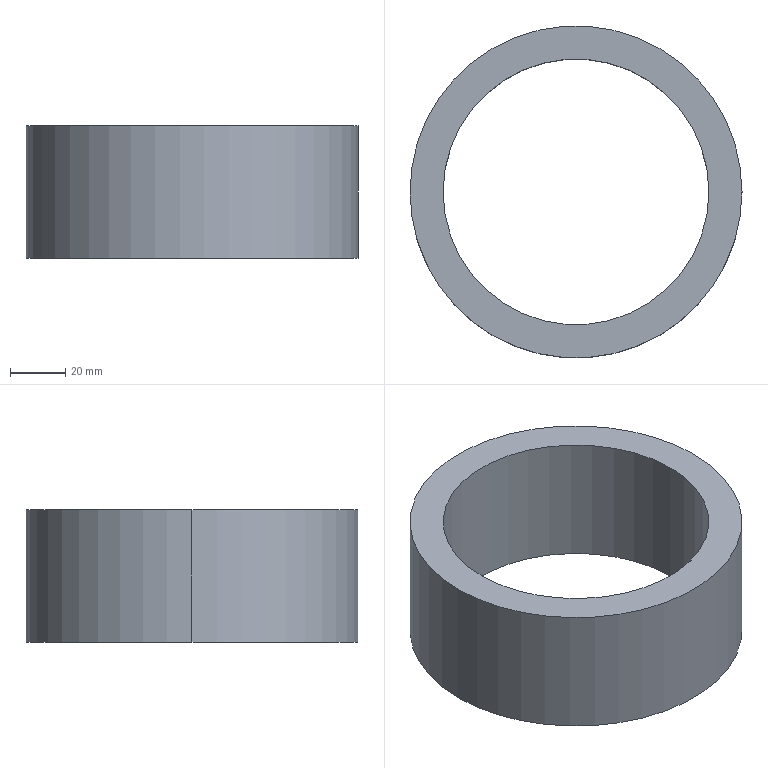Component | SolidWorks | 5-1 | 1 solid | 6 faces | box 120 x 120 x 48 mm | volume 194998 mm3 | cylinder 4 | plane 2 | commonest cylinder face diameters 96.06 x2 120 x2
STEP:
#1=CARTESIAN_POINT('',(1.891,0.,-1.89));
#2=VERTEX_POINT('',#1);
#3=CARTESIAN_POINT('',(1.891,0.,-3.78));
#4=VERTEX_POINT('',#3);
#5=CARTESIAN_POINT('',(1.891,0.,-1.89));
#6=DIRECTION('',(0.,0.,-1.));
#7=VECTOR('',#6,39.37);
#8=LINE('',#5,#7);
#9=EDGE_CURVE('',#2,#4,#8,.T.);
#10=ORIENTED_EDGE('',*,*,#9,.F.);
#11=CARTESIAN_POINT('',(-1.891,0.,-1.89));
#12=VERTEX_POINT('',#11);
#13=CARTESIAN_POINT('',(0.,0.,-1.89));
#14=DIRECTION('',(0.,0.,1.));
#15=DIRECTION('',(1.,0.,0.));
#16=AXIS2_PLACEMENT_3D('',#13,#14,#15);
#17=CIRCLE('',#16,1.891);
#18=EDGE_CURVE('',#2,#12,#17,.T.);
#19=ORIENTED_EDGE('',*,*,#18,.T.);
#20=CARTESIAN_POINT('',(-1.891,0.,-3.78));
#21=VERTEX_POINT('',#20);
#22=CARTESIAN_POINT('',(-1.891,0.,-1.89));
#23=DIRECTION('',(0.,0.,-1.));
#24=VECTOR('',#23,39.37);
#25=LINE('',#22,#24);
#26=EDGE_CURVE('',#12,#21,#25,.T.);
#27=ORIENTED_EDGE('',*,*,#26,.T.);
#28=CARTESIAN_POINT('',(0.,0.,-3.78));
#29=DIRECTION('',(0.,0.,1.));
#30=DIRECTION('',(1.,0.,0.));
#31=AXIS2_PLACEMENT_3D('',#28,#29,#30);
#32=CIRCLE('',#31,1.891);
#33=EDGE_CURVE('',#4,#21,#32,.T.);
#34=ORIENTED_EDGE('',*,*,#33,.F.);
#35=EDGE_LOOP('',(#10,#19,#27,#34));
#36=FACE_OUTER_BOUND('',#35,.T.);
#37=CARTESIAN_POINT('',(0.,0.,-1.89));
#38=DIRECTION('',(0.,0.,-1.));
#39=DIRECTION('',(-1.,0.,0.));
#40=AXIS2_PLACEMENT_3D('',#37,#38,#39);
#41=CYLINDRICAL_SURFACE('',#40,1.891);
#42=ADVANCED_FACE('',(#36),#41,.F.);
#43=CARTESIAN_POINT('',(2.362,0.,-1.89));
#44=VERTEX_POINT('',#43);
#45=CARTESIAN_POINT('',(2.362,0.,-3.78));
#46=VERTEX_POINT('',#45);
#47=CARTESIAN_POINT('',(2.362,0.,-1.89));
#48=DIRECTION('',(0.,0.,-1.));
#49=VECTOR('',#48,39.37);
#50=LINE('',#47,#49);
#51=EDGE_CURVE('',#44,#46,#50,.T.);
#52=ORIENTED_EDGE('',*,*,#51,.F.);
#53=CARTESIAN_POINT('',(-2.362,0.,-1.89));
#54=VERTEX_POINT('',#53);
#55=CARTESIAN_POINT('',(0.,0.,-1.89));
#56=DIRECTION('',(0.,0.,1.));
#57=DIRECTION('',(1.,0.,0.));
#58=AXIS2_PLACEMENT_3D('',#55,#56,#57);
#59=CIRCLE('',#58,2.362);
#60=EDGE_CURVE('',#54,#44,#59,.T.);
#61=ORIENTED_EDGE('',*,*,#60,.F.);
#62=CARTESIAN_POINT('',(-2.362,0.,-3.78));
#63=VERTEX_POINT('',#62);
#64=CARTESIAN_POINT('',(-2.362,0.,-1.89));
#65=DIRECTION('',(0.,0.,-1.));
#66=VECTOR('',#65,39.37);
#67=LINE('',#64,#66);
#68=EDGE_CURVE('',#54,#63,#67,.T.);
#69=ORIENTED_EDGE('',*,*,#68,.T.);
#70=CARTESIAN_POINT('',(0.,0.,-3.78));
#71=DIRECTION('',(0.,0.,1.));
#72=DIRECTION('',(1.,0.,0.));
#73=AXIS2_PLACEMENT_3D('',#70,#71,#72);
#74=CIRCLE('',#73,2.362);
#75=EDGE_CURVE('',#63,#46,#74,.T.);
#76=ORIENTED_EDGE('',*,*,#75,.T.);
#77=EDGE_LOOP('',(#52,#61,#69,#76));
#78=FACE_OUTER_BOUND('',#77,.T.);
#79=CARTESIAN_POINT('',(0.,0.,-1.89));
#80=DIRECTION('',(0.,0.,-1.));
#81=DIRECTION('',(-1.,0.,0.));
#82=AXIS2_PLACEMENT_3D('',#79,#80,#81);
#83=CYLINDRICAL_SURFACE('',#82,2.362);
#84=ADVANCED_FACE('',(#78),#83,.T.);
#85=CARTESIAN_POINT('',(0.,0.,-3.78));
#86=DIRECTION('',(0.,0.,1.));
#87=DIRECTION('',(1.,0.,0.));
#88=AXIS2_PLACEMENT_3D('',#85,#86,#87);
#89=CIRCLE('',#88,1.891);
#90=EDGE_CURVE('',#21,#4,#89,.T.);
#91=ORIENTED_EDGE('',*,*,#90,.T.);
#92=ORIENTED_EDGE('',*,*,#33,.T.);
#93=EDGE_LOOP('',(#91,#92));
#94=FACE_BOUND('',#93,.T.);
#95=ORIENTED_EDGE('',*,*,#75,.F.);
#96=CARTESIAN_POINT('',(0.,0.,-3.78));
#97=DIRECTION('',(0.,0.,1.));
#98=DIRECTION('',(1.,0.,0.));
#99=AXIS2_PLACEMENT_3D('',#96,#97,#98);
#100=CIRCLE('',#99,2.362);
#101=EDGE_CURVE('',#46,#63,#100,.T.);
#102=ORIENTED_EDGE('',*,*,#101,.F.);
#103=EDGE_LOOP('',(#95,#102));
#104=FACE_OUTER_BOUND('',#103,.T.);
#105=CARTESIAN_POINT('',(0.,0.,-3.78));
#106=DIRECTION('',(0.,0.,1.));
#107=DIRECTION('',(1.,0.,0.));
#108=AXIS2_PLACEMENT_3D('',#105,#106,#107);
#109=PLANE('',#108);
#110=ADVANCED_FACE('',(#94,#104),#109,.F.);
#111=CARTESIAN_POINT('',(0.,0.,-1.89));
#112=DIRECTION('',(0.,0.,1.));
#113=DIRECTION('',(1.,0.,0.));
#114=AXIS2_PLACEMENT_3D('',#111,#112,#113);
#115=CIRCLE('',#114,1.891);
#116=EDGE_CURVE('',#12,#2,#115,.T.);
#117=ORIENTED_EDGE('',*,*,#116,.F.);
#118=ORIENTED_EDGE('',*,*,#18,.F.);
#119=EDGE_LOOP('',(#117,#118));
#120=FACE_BOUND('',#119,.T.);
#121=ORIENTED_EDGE('',*,*,#60,.T.);
#122=CARTESIAN_POINT('',(0.,0.,-1.89));
#123=DIRECTION('',(0.,0.,1.));
#124=DIRECTION('',(1.,0.,0.));
#125=AXIS2_PLACEMENT_3D('',#122,#123,#124);
#126=CIRCLE('',#125,2.362);
#127=EDGE_CURVE('',#44,#54,#126,.T.);
#128=ORIENTED_EDGE('',*,*,#127,.T.);
#129=EDGE_LOOP('',(#121,#128));
#130=FACE_OUTER_BOUND('',#129,.T.);
#131=CARTESIAN_POINT('',(0.,0.,-1.89));
#132=DIRECTION('',(0.,0.,1.));
#133=DIRECTION('',(1.,0.,0.));
#134=AXIS2_PLACEMENT_3D('',#131,#132,#133);
#135=PLANE('',#134);
#136=ADVANCED_FACE('',(#120,#130),#135,.T.);
#137=ORIENTED_EDGE('',*,*,#127,.F.);
#138=ORIENTED_EDGE('',*,*,#51,.T.);
#139=ORIENTED_EDGE('',*,*,#101,.T.);
#140=ORIENTED_EDGE('',*,*,#68,.F.);
#141=EDGE_LOOP('',(#137,#138,#139,#140));
#142=FACE_OUTER_BOUND('',#141,.T.);
#143=CARTESIAN_POINT('',(0.,0.,-1.89));
#144=DIRECTION('',(0.,0.,-1.));
#145=DIRECTION('',(-1.,0.,0.));
#146=AXIS2_PLACEMENT_3D('',#143,#144,#145);
#147=CYLINDRICAL_SURFACE('',#146,2.362);
#148=ADVANCED_FACE('',(#142),#147,.T.);
#149=ORIENTED_EDGE('',*,*,#116,.T.);
#150=ORIENTED_EDGE('',*,*,#9,.T.);
#151=ORIENTED_EDGE('',*,*,#90,.F.);
#152=ORIENTED_EDGE('',*,*,#26,.F.);
#153=EDGE_LOOP('',(#149,#150,#151,#152));
#154=FACE_OUTER_BOUND('',#153,.T.);
#155=CARTESIAN_POINT('',(0.,0.,-1.89));
#156=DIRECTION('',(0.,0.,-1.));
#157=DIRECTION('',(-1.,0.,0.));
#158=AXIS2_PLACEMENT_3D('',#155,#156,#157);
#159=CYLINDRICAL_SURFACE('',#158,1.891);
#160=ADVANCED_FACE('',(#154),#159,.F.);
#161=CLOSED_SHELL('',(#42,#84,#110,#136,#148,#160));
#162=MANIFOLD_SOLID_BREP('',#161);
#163=CARTESIAN_POINT('',(0.,0.,0.));
#164=DIRECTION('',(0.,0.,1.));
#165=DIRECTION('',(1.,0.,0.));
#166=AXIS2_PLACEMENT_3D('',#163,#164,#165);
#167=(LENGTH_UNIT()NAMED_UNIT(*)SI_UNIT($,.METRE.));
#168=LENGTH_MEASURE_WITH_UNIT(LENGTH_MEASURE(0.0254),#167);
#169=DIMENSIONAL_EXPONENTS(1.,0.,0.,0.,0.,0.,0.);
#170=(CONVERSION_BASED_UNIT('',#168)LENGTH_UNIT()NAMED_UNIT(#169));
#171=UNCERTAINTY_MEASURE_WITH_UNIT(LENGTH_MEASURE(0.00001),#170,'','');
#172=(NAMED_UNIT(*)PLANE_ANGLE_UNIT()SI_UNIT($,.RADIAN.));
#173=(NAMED_UNIT(*)SI_UNIT($,.STERADIAN.)SOLID_ANGLE_UNIT());
#174=(GEOMETRIC_REPRESENTATION_CONTEXT(3)GLOBAL_UNCERTAINTY_ASSIGNED_CONTEXT((#171))GLOBAL_UNIT_ASSIGNED_CONTEXT((#170,#172,#173))REPRESENTATION_CONTEXT('',''));
#175=ADVANCED_BREP_SHAPE_REPRESENTATION('',(#162,#166),#174);
#176=COLOUR_RGB('',0.7922,0.8196,0.9333);
#177=FILL_AREA_STYLE_COLOUR('',#176);
#178=FILL_AREA_STYLE('',(#177));
#179=SURFACE_STYLE_FILL_AREA(#178);
#180=SURFACE_SIDE_STYLE('',(#179));
#181=SURFACE_STYLE_USAGE(.BOTH.,#180);
#182=PRESENTATION_STYLE_ASSIGNMENT((#181));
#183=STYLED_ITEM('',(#182),#162);
#184=PRESENTATION_LAYER_ASSIGNMENT('','',(#183));
#185=(LENGTH_UNIT()NAMED_UNIT(*)SI_UNIT($,.METRE.));
#186=LENGTH_MEASURE_WITH_UNIT(LENGTH_MEASURE(0.0254),#185);
#187=DIMENSIONAL_EXPONENTS(1.,0.,0.,0.,0.,0.,0.);
#188=(CONVERSION_BASED_UNIT('',#186)LENGTH_UNIT()NAMED_UNIT(#187));
#189=UNCERTAINTY_MEASURE_WITH_UNIT(LENGTH_MEASURE(0.00001),#188,'','');
#190=(NAMED_UNIT(*)PLANE_ANGLE_UNIT()SI_UNIT($,.RADIAN.));
#191=(NAMED_UNIT(*)SI_UNIT($,.STERADIAN.)SOLID_ANGLE_UNIT());
#192=(GEOMETRIC_REPRESENTATION_CONTEXT(3)GLOBAL_UNCERTAINTY_ASSIGNED_CONTEXT((#189))GLOBAL_UNIT_ASSIGNED_CONTEXT((#188,#190,#191))REPRESENTATION_CONTEXT('',''));
#193=MECHANICAL_DESIGN_GEOMETRIC_PRESENTATION_REPRESENTATION('',(#183),#192);